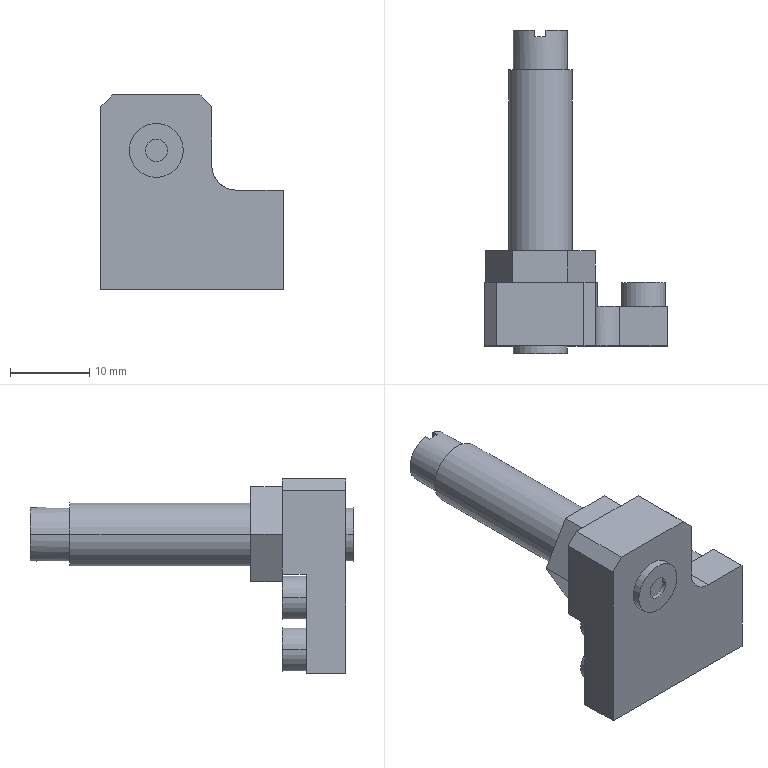Component | SolidWorks | MXQ8-30B-M9N_0_0_MXQ8-30B-M9N_0_0-2_MXQ8-30B-M9N_0_0_4_20-1 | 1 solid | 78 faces | volume 4858 mm3 | plane 61 | cylinder 17 | commonest cylinder face diameters 5.5 x8 6.8 x4 2.8 x2 8 x2 6 x1